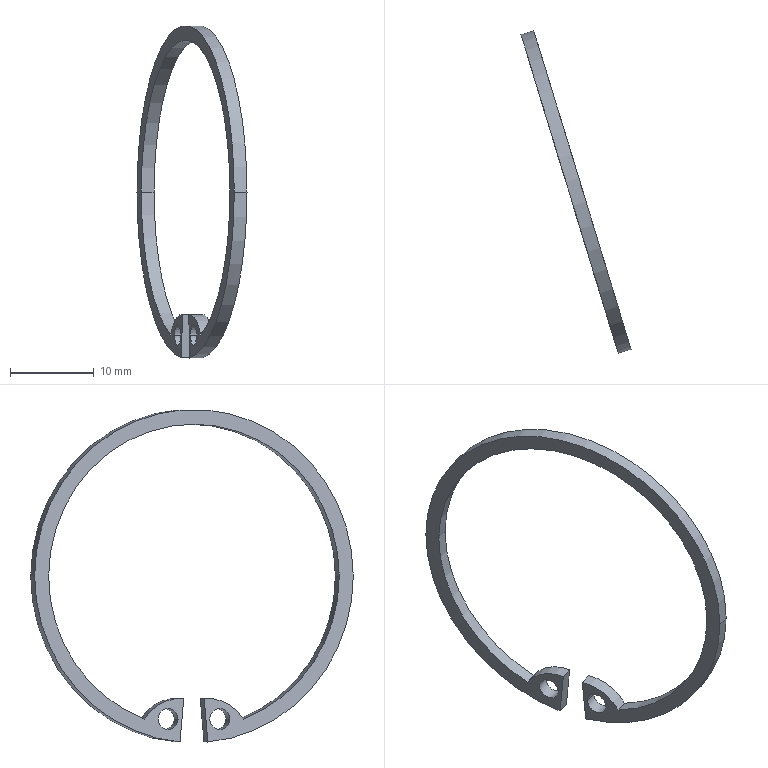Component | SolidWorks | v1ZHXTBGMWB6904ZZ_40SB1-1_v1ZHXTRRING37SB1-1 | 1 solid | 16 faces | box 13.15 x 38.53 x 39.72 mm | volume 346 mm3 | cylinder 12 | plane 4 | commonest cylinder face diameters 2.5 x4 36.3 x3 39.8 x3 10.4 x2
build123d program:
from build123d import *

# Parameters (mm, degrees)
SKETCH1_R           = 1.25
BOSS_EXTRUDE1_DEPTH = 1.6


with BuildPart() as part:
    # Sketch1 → Boss-Extrude1 (new body)
    with BuildSketch(Plane.XY):
        with BuildLine():
            Line((-1.734, -19.824), (-1.281, -14.644))
            ThreePointArc((-1.281, -14.644), (-4.059, -15.173), (-6.149, -17.077))
            ThreePointArc((-6.149, -17.077), (0, 18.15), (6.149, -17.077))
            ThreePointArc((6.149, -17.077), (4.059, -15.173), (1.281, -14.644))
            Line((1.281, -14.644), (1.734, -19.824))
            ThreePointArc((1.734, -19.824), (0, 19.9), (-1.734, -19.824))
        make_face()
        with Locations((3.235, -17.083)):
            Circle(SKETCH1_R, mode=Mode.SUBTRACT)
        with Locations((-3.235, -17.083)):
            Circle(SKETCH1_R, mode=Mode.SUBTRACT)
    extrude(amount=BOSS_EXTRUDE1_DEPTH)


solid = part.part

# Placed as in the assembly
solid = solid.moved(Location((156.058, -238.604, 375.239), (-90, 73.032, -180)))